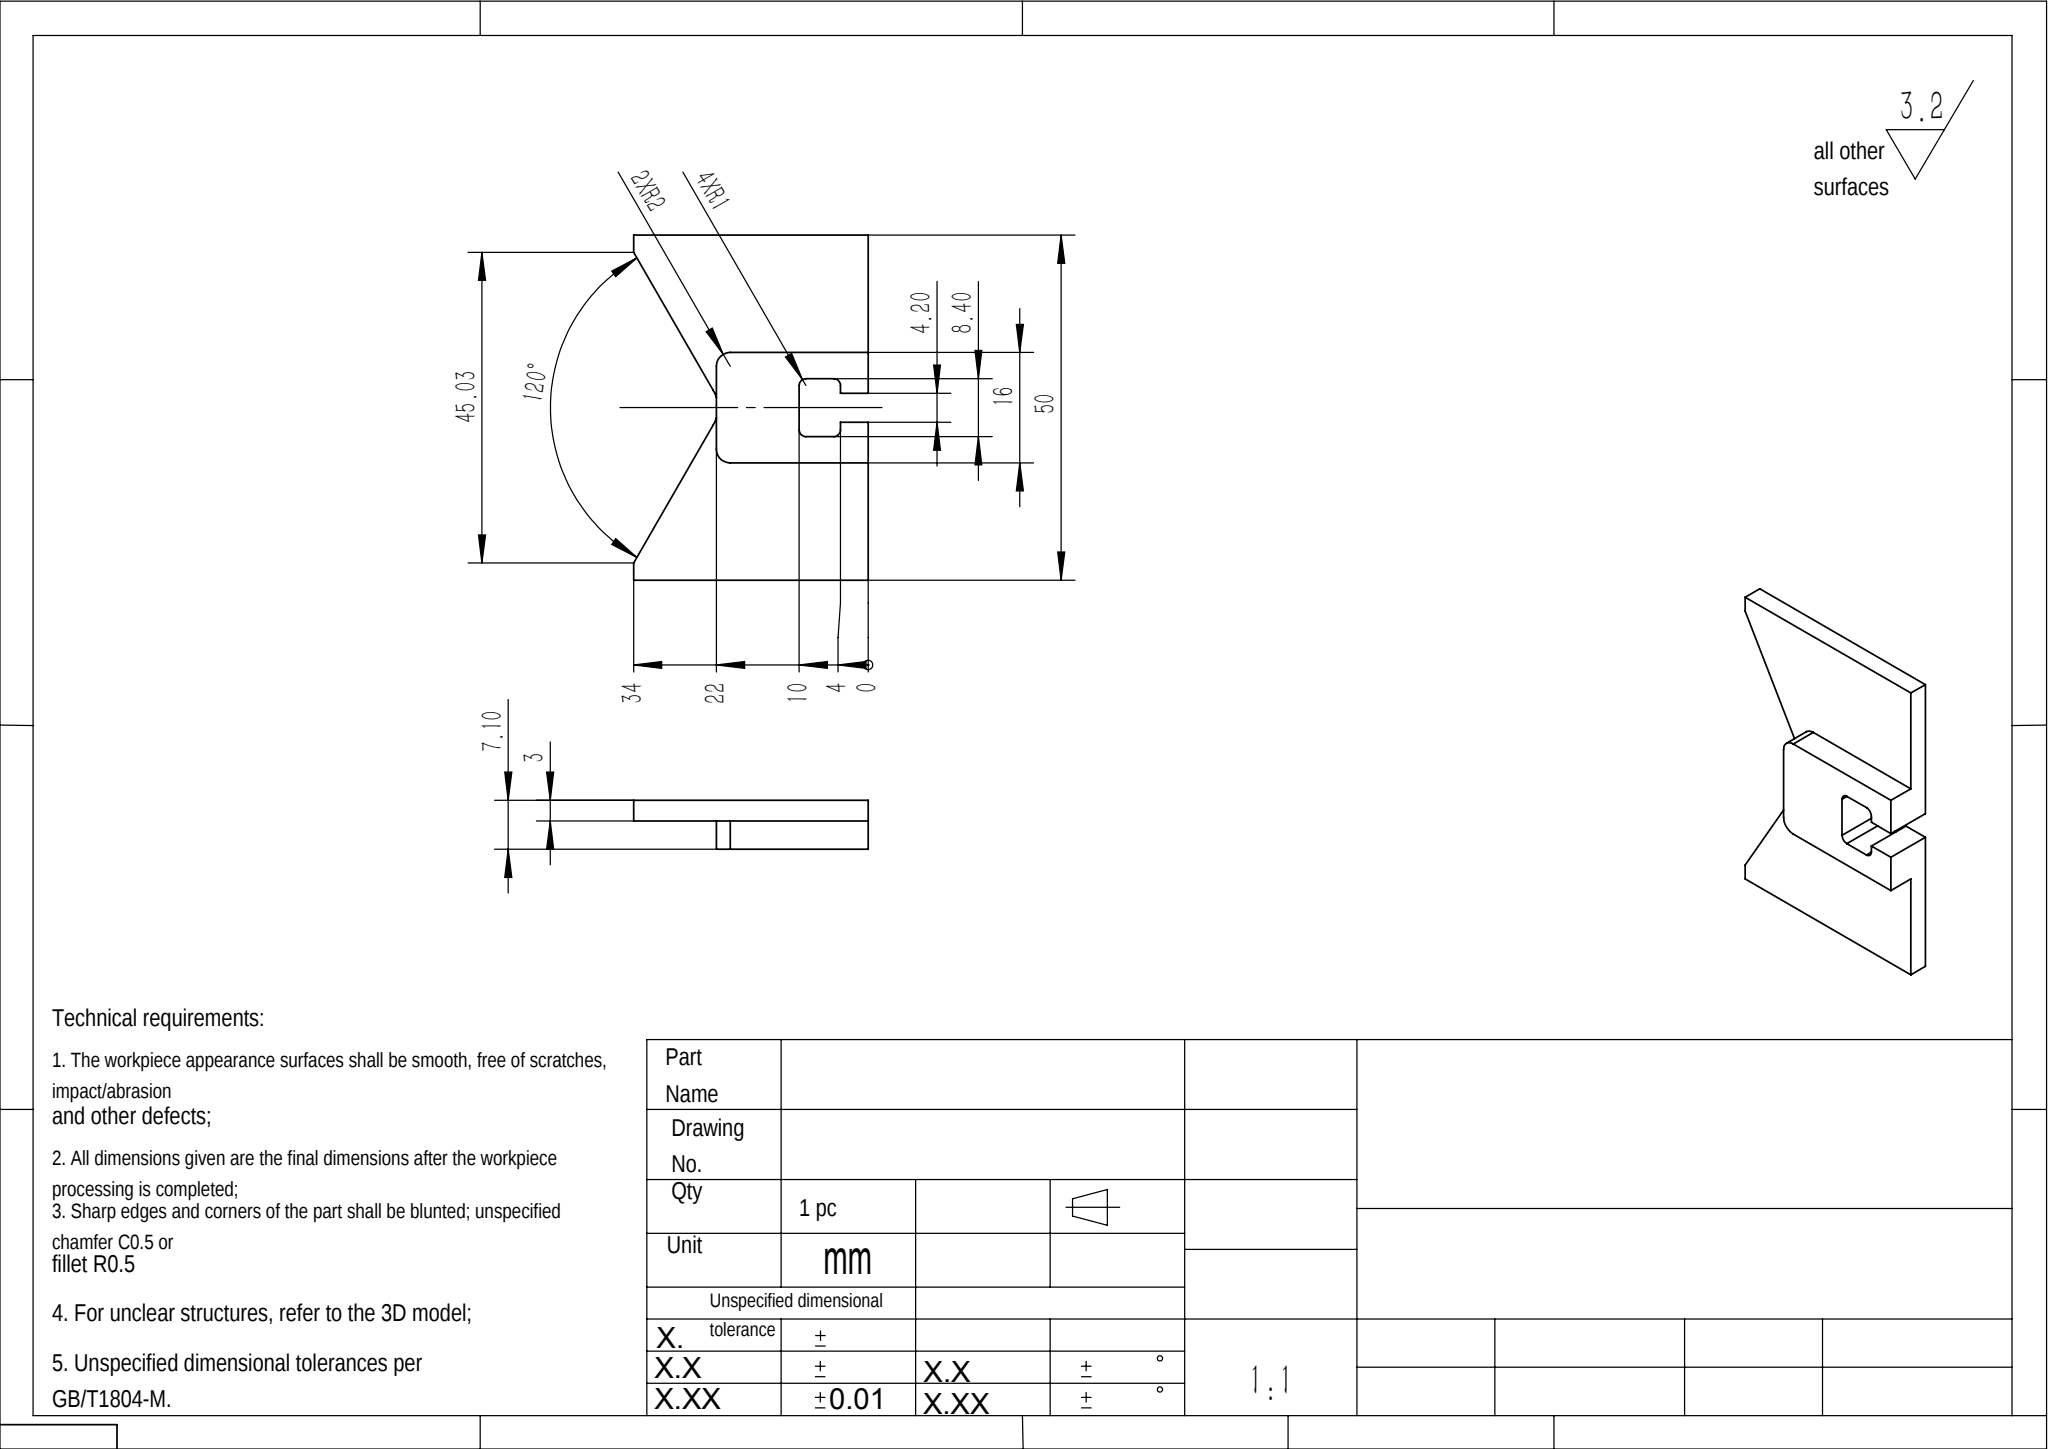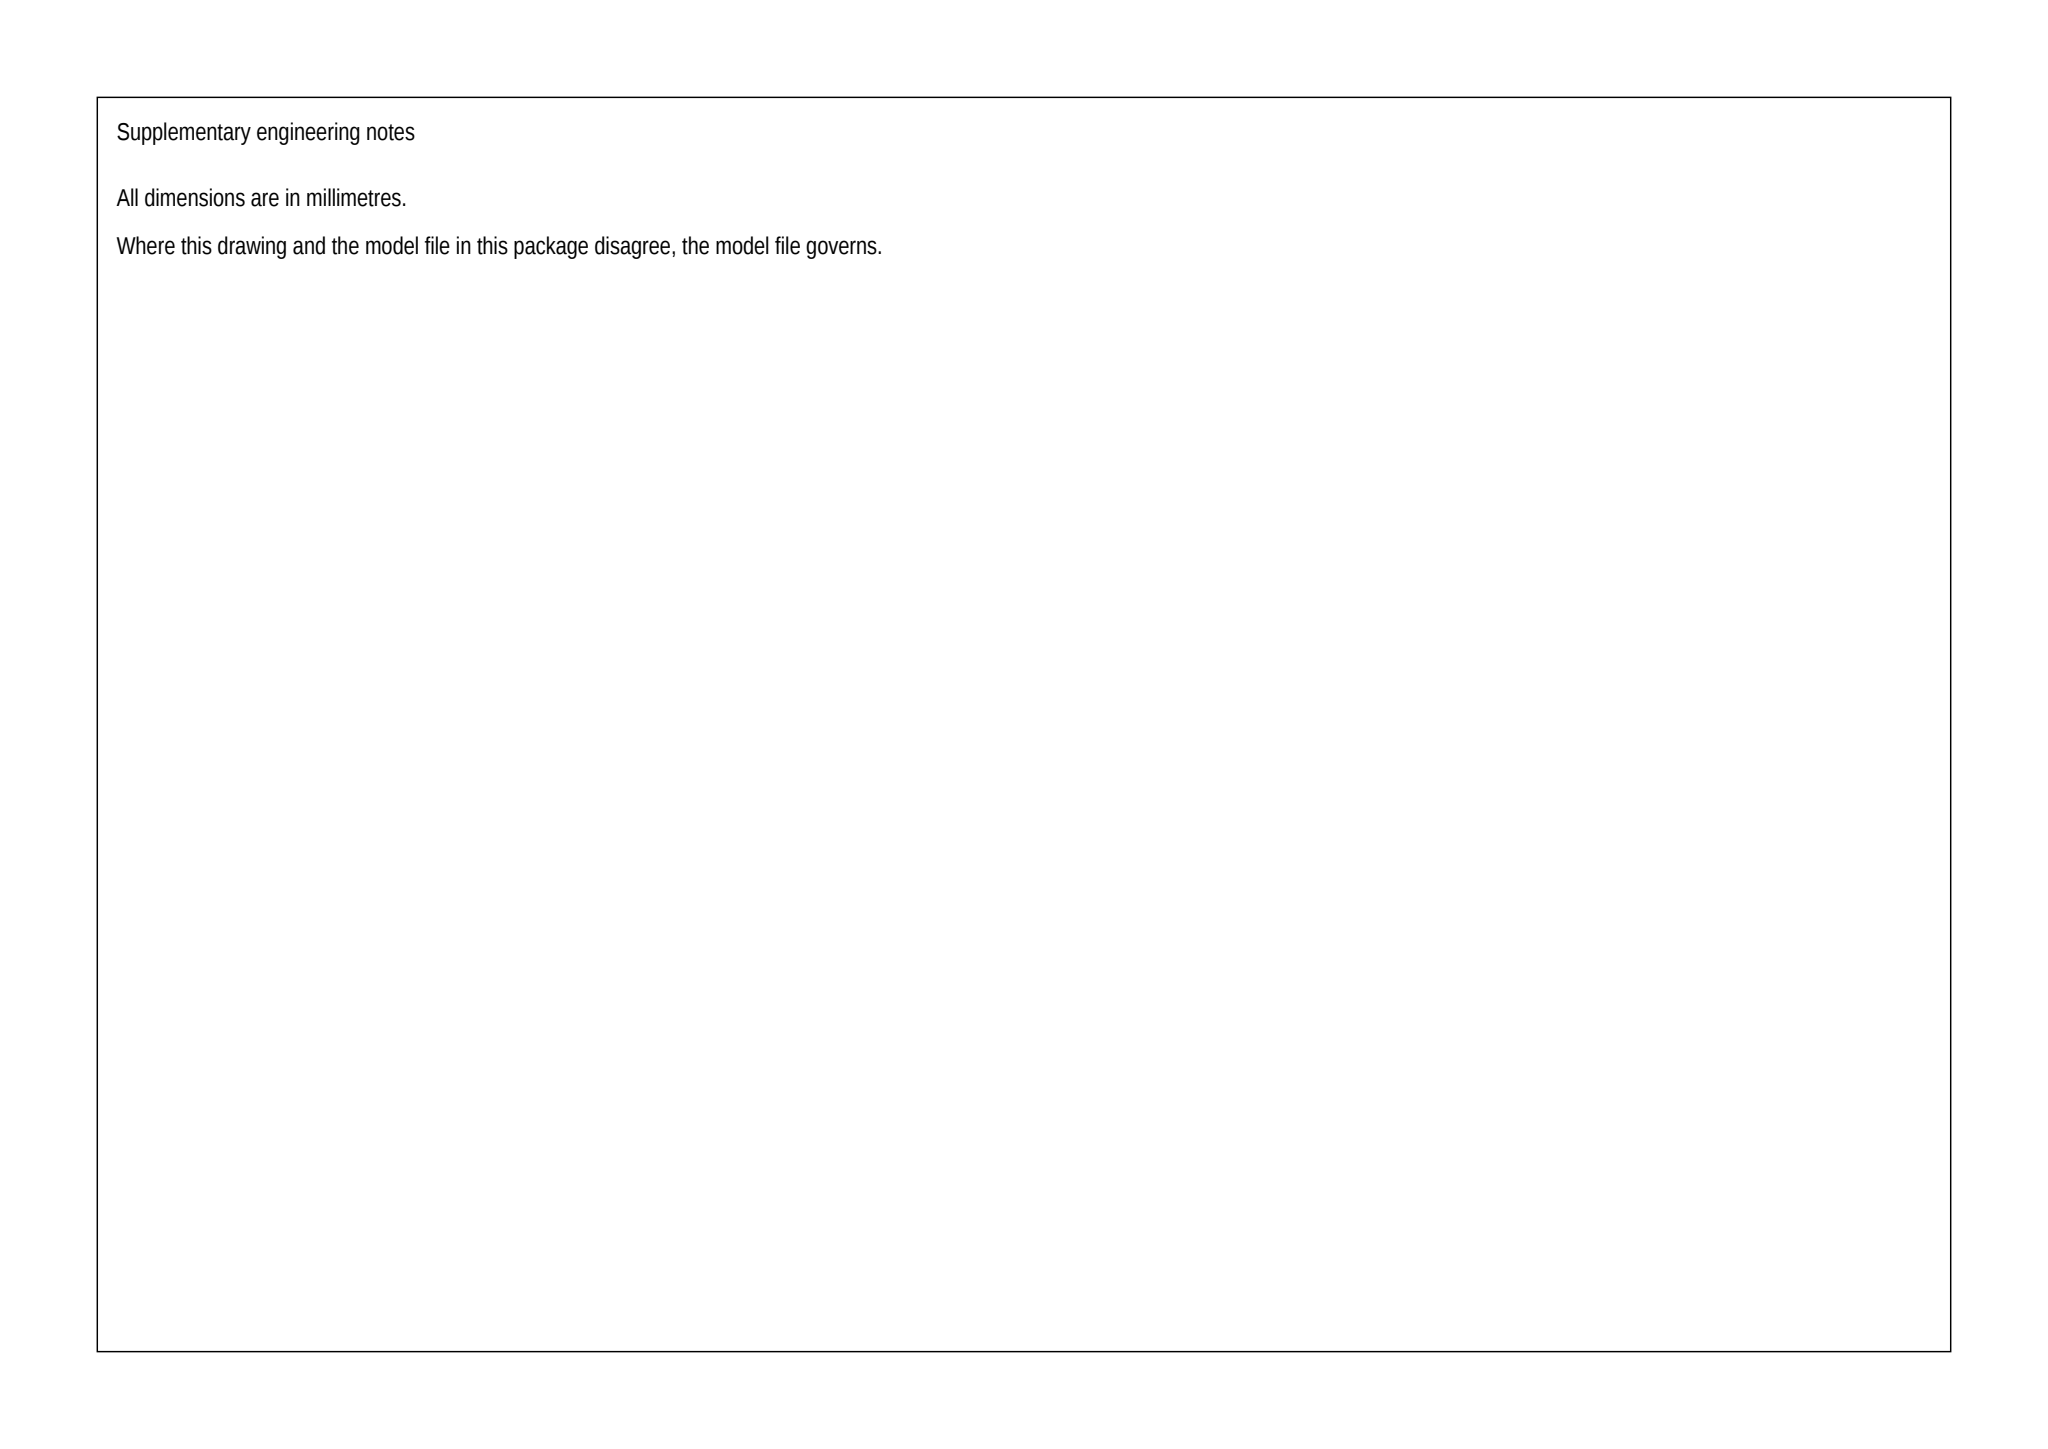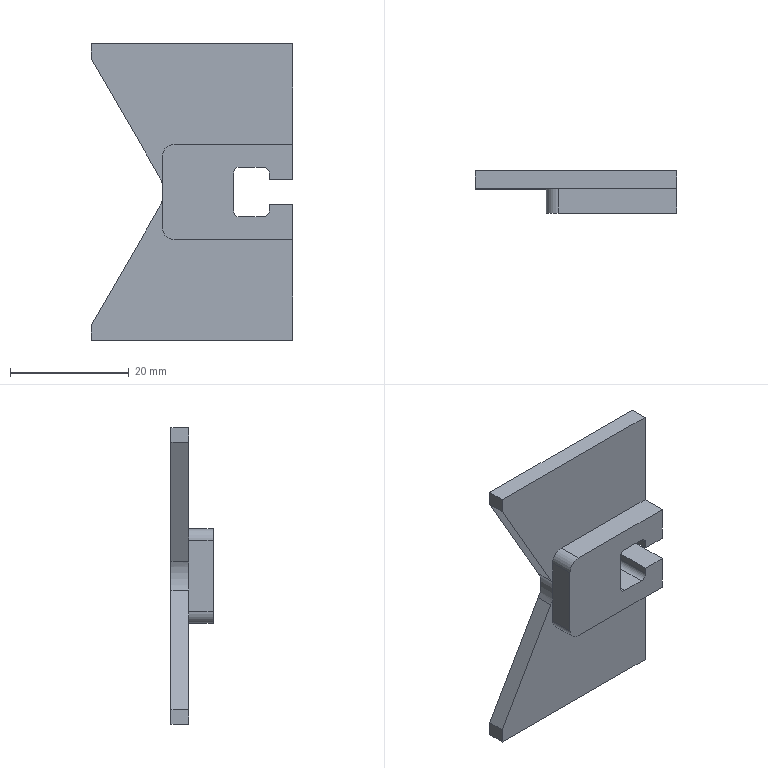Part | SolidWorks | mm | 1 solid | 30 faces | box 34 x 7.1 x 50 mm | volume 5191 mm3 | plane 23 | cylinder 7 | commonest cylinder face diameters 2 x4 4 x2 10 x1
build123d program:
from build123d import *

# Parameters (mm, degrees)
BOSS_EXTRUDE1_DEPTH = 3
FILLET1_R           = 5
SKETCH2_W           = 22
SKETCH2_H           = 16
BOSS_EXTRUDE2_DEPTH = 4.1
FILLET2_R           = 2
CUT_EXTRUDE1_DEPTH  = 20
FILLET3_R           = 1


with BuildPart() as part:
    # Sketch1 → Boss-Extrude1 (new body)
    with BuildSketch(Plane(origin=(0, 0, 0), x_dir=(1, 0, 0), z_dir=(0, 1, 0))):
        Polygon((0, 25), (0, -25), (-34, -25), (-34, -22.517), (-21, 0), (-34, 22.517), (-34, 25), align=None)
    extrude(amount=BOSS_EXTRUDE1_DEPTH)

    # Fillet1
    fillet1_edges = [part.edges().sort_by_distance(p)[0] for p in [
        (-21, 1.5, 0),
    ]]
    fillet(fillet1_edges, radius=FILLET1_R)

    # Sketch2 → Boss-Extrude2 (add)
    with BuildSketch(Plane.XZ):
        with Locations((-11, 0)):
            Rectangle(SKETCH2_W, SKETCH2_H)
    extrude(amount=BOSS_EXTRUDE2_DEPTH)

    # Fillet2
    fillet2_edges = [part.edges().sort_by_distance(p)[0] for p in [
        (-22, -2.05, 8),
        (-22, -2.05, -8),
    ]]
    fillet(fillet2_edges, radius=FILLET2_R)

    # Sketch3 → Cut-Extrude1 (cut)
    with BuildSketch(Plane(origin=(0, 3, 0), x_dir=(1, 0, 0), z_dir=(0, 1, 0))):
        Polygon((-4, 4.2), (-4, 2.1), (0, 2.1), (0, -2.1), (-4, -2.1), (-4, -4.2), (-10, -4.2), (-10, 4.2), align=None)
    extrude(amount=-CUT_EXTRUDE1_DEPTH, mode=Mode.SUBTRACT)

    # Fillet3
    fillet3_edges = [part.edges().sort_by_distance(p)[0] for p in [
        (-10, -0.55, -4.2),
        (-4, -0.55, -4.2),
        (-4, -0.55, 4.2),
        (-10, -0.55, 4.2),
    ]]
    fillet(fillet3_edges, radius=FILLET3_R)


solid = part.part